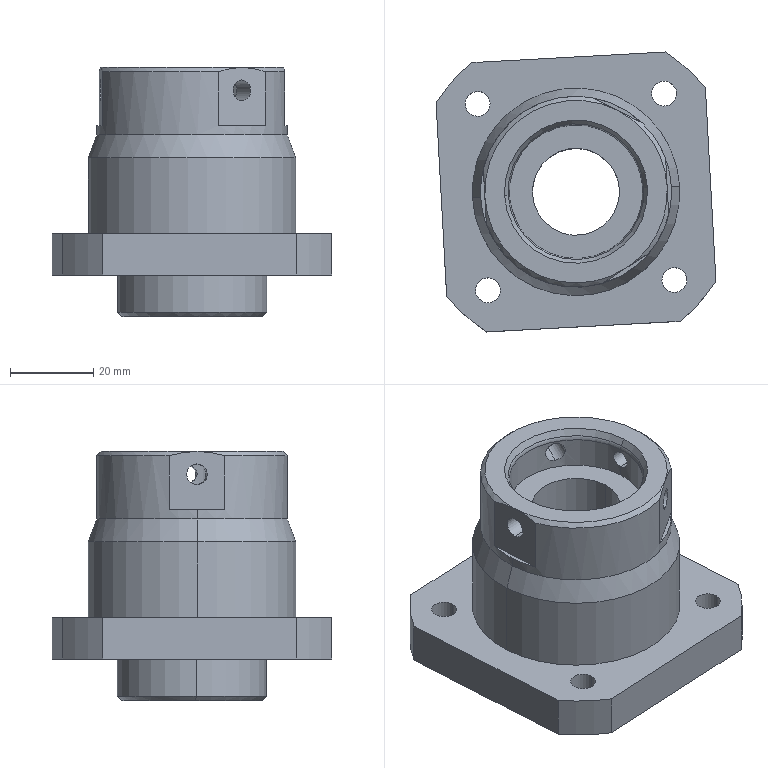Component | SolidWorks | T160418-M01U03-P08-1 | 1 solid | 61 faces | volume 95933 mm3 | cylinder 30 | plane 17 | cone 12 | torus 2 | commonest cylinder face diameters 6 x8 5 x6 80 x4 4.2 x2 32.2 x2 46 x2 50 x2 36 x2 | material SKS3